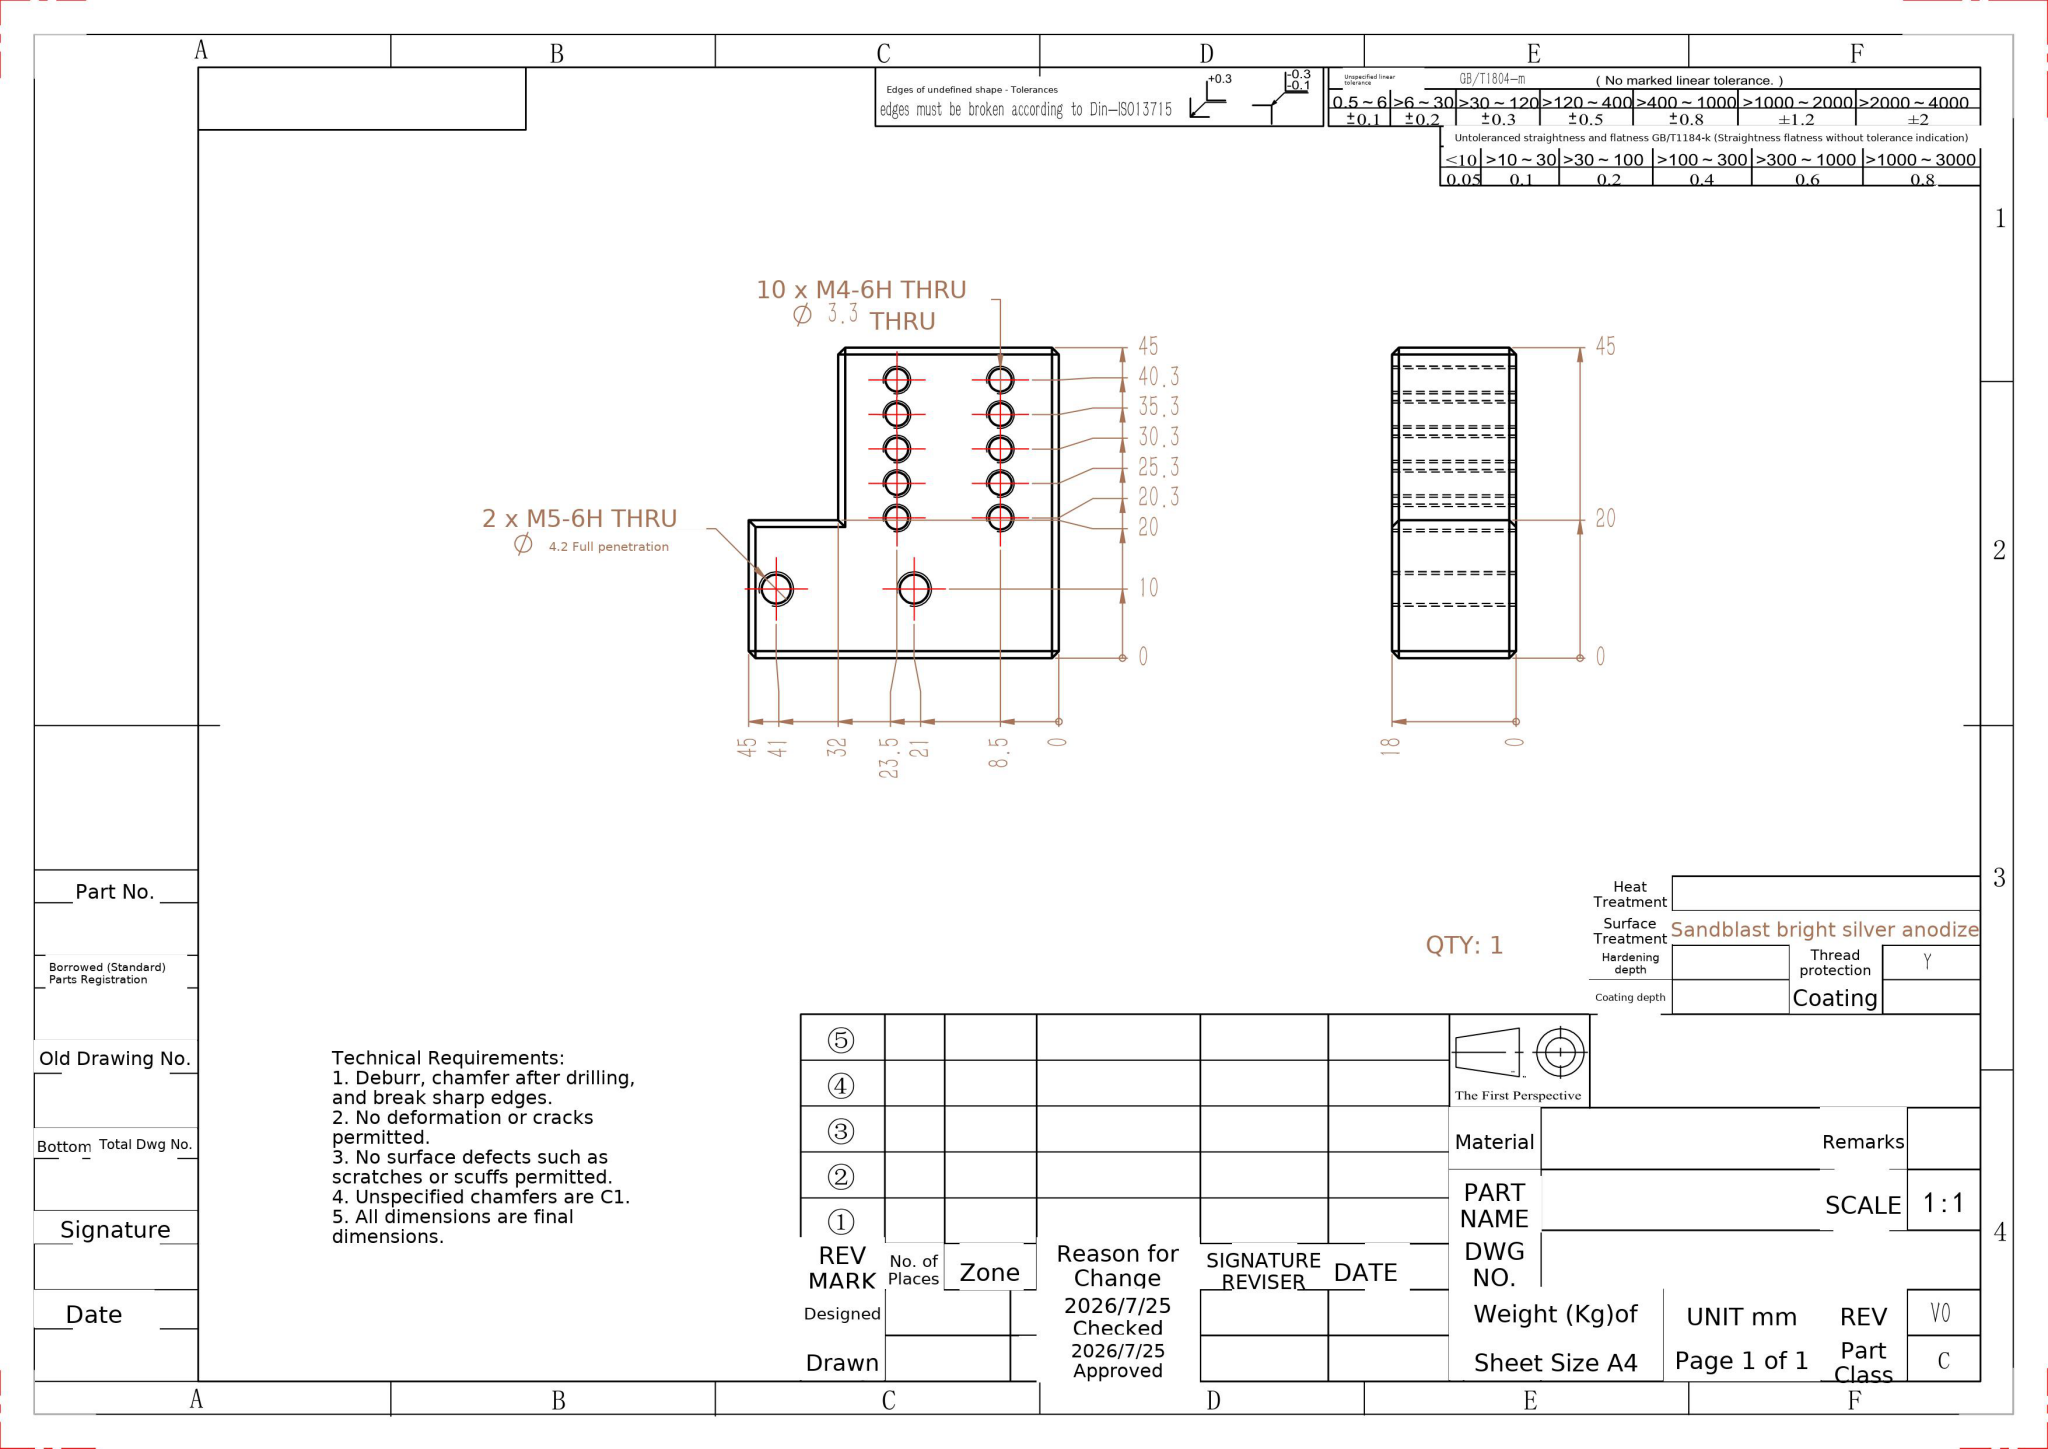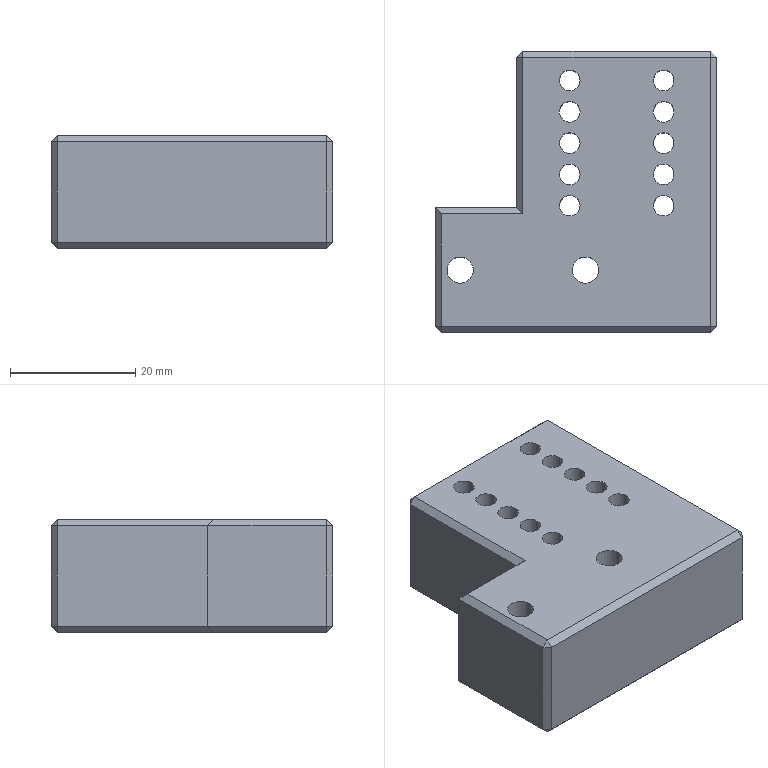Part | NX | mm | 1 solid | 56 faces | box 45 x 45 x 18 mm | volume 28351 mm3 | plane 32 | cylinder 24 | commonest cylinder face diameters 3.3 x20 4.2 x4